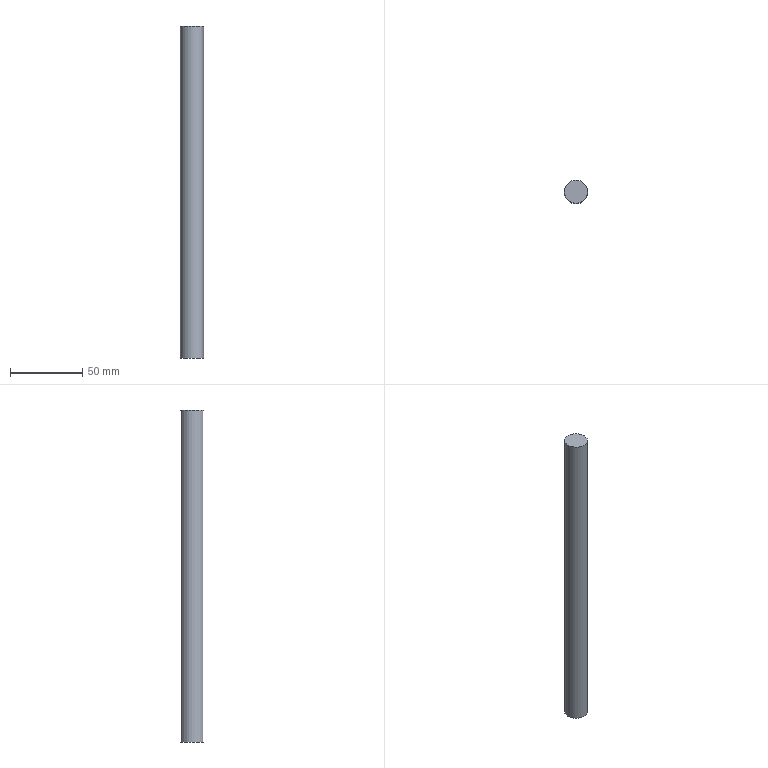Component | NX | STUD_A | 1 solid | 3 faces | box 16 x 16 x 230 mm | volume 46244 mm3 | plane 2 | cylinder 1 | commonest cylinder face diameters 16 x1
STEP:
#1=CARTESIAN_POINT('',(0.,0.,0.));
#2=DIRECTION('',(0.,0.,1.));
#3=DIRECTION('',(1.,0.,0.));
#4=AXIS2_PLACEMENT_3D('',#1,#2,#3);
#5=CARTESIAN_POINT('',(-119.,0.,240.));
#6=VERTEX_POINT('',#5);
#7=CARTESIAN_POINT('',(-111.,0.,240.));
#8=DIRECTION('',(0.,0.,-1.));
#9=DIRECTION('',(-1.,0.,0.));
#10=AXIS2_PLACEMENT_3D('',#7,#8,#9);
#11=CIRCLE('',#10,8.);
#12=CARTESIAN_POINT('',(-111.,0.,240.));
#13=DIRECTION('',(0.,0.,1.));
#14=DIRECTION('',(-1.,0.,0.));
#15=AXIS2_PLACEMENT_3D('',#12,#13,#14);
#16=PLANE('',#15);
#17=CARTESIAN_POINT('',(8.,0.));
#18=CARTESIAN_POINT('',(8.,-13.856));
#19=CARTESIAN_POINT('',(-4.,-6.928));
#20=CARTESIAN_POINT('',(-16.,-0.));
#21=CARTESIAN_POINT('',(-4.,6.928));
#22=CARTESIAN_POINT('',(8.,13.856));
#23=CARTESIAN_POINT('',(8.,0.));
#24=(BOUNDED_CURVE()B_SPLINE_CURVE(2,(#17,#18,#19,#20,#21,#22,#23),.UNSPECIFIED.,.T.,.F.)B_SPLINE_CURVE_WITH_KNOTS((1,2,2,2,2,1),(-2.094,0.,2.094,4.189,6.283,8.378),.UNSPECIFIED.)CURVE()GEOMETRIC_REPRESENTATION_ITEM()RATIONAL_B_SPLINE_CURVE((1.,0.5,1.,0.5,1.,0.5,1.))REPRESENTATION_ITEM(''));
#25=(GEOMETRIC_REPRESENTATION_CONTEXT(2)PARAMETRIC_REPRESENTATION_CONTEXT()REPRESENTATION_CONTEXT('',''));
#26=DEFINITIONAL_REPRESENTATION('',(#24),#25);
#27=PCURVE('',#16,#26);
#28=CARTESIAN_POINT('',(-111.,0.,10.));
#29=DIRECTION('',(0.,0.,1.));
#30=DIRECTION('',(-1.,0.,0.));
#31=AXIS2_PLACEMENT_3D('',#28,#29,#30);
#32=CYLINDRICAL_SURFACE('',#31,8.);
#33=CARTESIAN_POINT('',(6.283,230.));
#34=DIRECTION('',(-1.,0.));
#35=VECTOR('',#34,1.);
#36=LINE('',#33,#35);
#37=(GEOMETRIC_REPRESENTATION_CONTEXT(2)PARAMETRIC_REPRESENTATION_CONTEXT()REPRESENTATION_CONTEXT('',''));
#38=DEFINITIONAL_REPRESENTATION('',(#36),#37);
#39=PCURVE('',#32,#38);
#40=SURFACE_CURVE('',#11,(#27,#39),.PCURVE_S1.);
#41=EDGE_CURVE('',#6,#6,#40,.T.);
#42=ORIENTED_EDGE('',*,*,#41,.F.);
#43=EDGE_LOOP('',(#42));
#44=FACE_BOUND('',#43,.T.);
#45=ADVANCED_FACE('',(#44),#16,.T.);
#46=CARTESIAN_POINT('',(-119.,0.,10.));
#47=VERTEX_POINT('',#46);
#48=CARTESIAN_POINT('',(-111.,0.,10.));
#49=DIRECTION('',(0.,0.,1.));
#50=DIRECTION('',(-1.,0.,0.));
#51=AXIS2_PLACEMENT_3D('',#48,#49,#50);
#52=CIRCLE('',#51,8.);
#53=CARTESIAN_POINT('',(-111.,0.,10.));
#54=DIRECTION('',(0.,0.,-1.));
#55=DIRECTION('',(1.,0.,0.));
#56=AXIS2_PLACEMENT_3D('',#53,#54,#55);
#57=PLANE('',#56);
#58=CARTESIAN_POINT('',(-8.,0.));
#59=CARTESIAN_POINT('',(-8.,13.856));
#60=CARTESIAN_POINT('',(4.,6.928));
#61=CARTESIAN_POINT('',(16.,0.));
#62=CARTESIAN_POINT('',(4.,-6.928));
#63=CARTESIAN_POINT('',(-8.,-13.856));
#64=CARTESIAN_POINT('',(-8.,0.));
#65=(BOUNDED_CURVE()B_SPLINE_CURVE(2,(#58,#59,#60,#61,#62,#63,#64),.UNSPECIFIED.,.T.,.F.)B_SPLINE_CURVE_WITH_KNOTS((1,2,2,2,2,1),(-2.094,0.,2.094,4.189,6.283,8.378),.UNSPECIFIED.)CURVE()GEOMETRIC_REPRESENTATION_ITEM()RATIONAL_B_SPLINE_CURVE((1.,0.5,1.,0.5,1.,0.5,1.))REPRESENTATION_ITEM(''));
#66=(GEOMETRIC_REPRESENTATION_CONTEXT(2)PARAMETRIC_REPRESENTATION_CONTEXT()REPRESENTATION_CONTEXT('',''));
#67=DEFINITIONAL_REPRESENTATION('',(#65),#66);
#68=PCURVE('',#57,#67);
#69=CARTESIAN_POINT('',(0.,0.));
#70=DIRECTION('',(1.,0.));
#71=VECTOR('',#70,1.);
#72=LINE('',#69,#71);
#73=(GEOMETRIC_REPRESENTATION_CONTEXT(2)PARAMETRIC_REPRESENTATION_CONTEXT()REPRESENTATION_CONTEXT('',''));
#74=DEFINITIONAL_REPRESENTATION('',(#72),#73);
#75=PCURVE('',#32,#74);
#76=SURFACE_CURVE('',#52,(#68,#75),.PCURVE_S1.);
#77=EDGE_CURVE('',#47,#47,#76,.T.);
#78=ORIENTED_EDGE('',*,*,#77,.F.);
#79=EDGE_LOOP('',(#78));
#80=FACE_BOUND('',#79,.T.);
#81=ADVANCED_FACE('',(#80),#57,.T.);
#82=ORIENTED_EDGE('',*,*,#41,.T.);
#83=CARTESIAN_POINT('',(-119.,0.,10.));
#84=CARTESIAN_POINT('',(-119.,0.,240.));
#85=B_SPLINE_CURVE_WITH_KNOTS('',1,(#83,#84),.UNSPECIFIED.,.F.,.F.,(2,2),(0.,230.),.PIECEWISE_BEZIER_KNOTS.);
#86=CARTESIAN_POINT('',(0.,0.));
#87=DIRECTION('',(0.,1.));
#88=VECTOR('',#87,1.);
#89=LINE('',#86,#88);
#90=(GEOMETRIC_REPRESENTATION_CONTEXT(2)PARAMETRIC_REPRESENTATION_CONTEXT()REPRESENTATION_CONTEXT('',''));
#91=DEFINITIONAL_REPRESENTATION('',(#89),#90);
#92=PCURVE('',#32,#91);
#93=CARTESIAN_POINT('',(6.283,0.));
#94=DIRECTION('',(0.,1.));
#95=VECTOR('',#94,1.);
#96=LINE('',#93,#95);
#97=(GEOMETRIC_REPRESENTATION_CONTEXT(2)PARAMETRIC_REPRESENTATION_CONTEXT()REPRESENTATION_CONTEXT('',''));
#98=DEFINITIONAL_REPRESENTATION('',(#96),#97);
#99=PCURVE('',#32,#98);
#100=SEAM_CURVE('',#85,(#92,#99),.PCURVE_S1.);
#101=EDGE_CURVE('',#47,#6,#100,.T.);
#102=ORIENTED_EDGE('',*,*,#101,.F.);
#103=ORIENTED_EDGE('',*,*,#77,.T.);
#104=ORIENTED_EDGE('',*,*,#101,.T.);
#105=EDGE_LOOP('',(#82,#102,#103,#104));
#106=FACE_BOUND('',#105,.T.);
#107=ADVANCED_FACE('',(#106),#32,.T.);
#108=CLOSED_SHELL('',(#45,#81,#107));
#109=MANIFOLD_SOLID_BREP('',#108);
#110=(LENGTH_UNIT()NAMED_UNIT(*)SI_UNIT(.MILLI.,.METRE.));
#111=UNCERTAINTY_MEASURE_WITH_UNIT(LENGTH_MEASURE(0.00001),#110,'','');
#112=(NAMED_UNIT(*)PLANE_ANGLE_UNIT()SI_UNIT($,.RADIAN.));
#113=(NAMED_UNIT(*)SI_UNIT($,.STERADIAN.)SOLID_ANGLE_UNIT());
#114=(GEOMETRIC_REPRESENTATION_CONTEXT(3)GLOBAL_UNCERTAINTY_ASSIGNED_CONTEXT((#111))GLOBAL_UNIT_ASSIGNED_CONTEXT((#110,#112,#113))REPRESENTATION_CONTEXT('',''));
#115=ADVANCED_BREP_SHAPE_REPRESENTATION('',(#4,#109),#114);